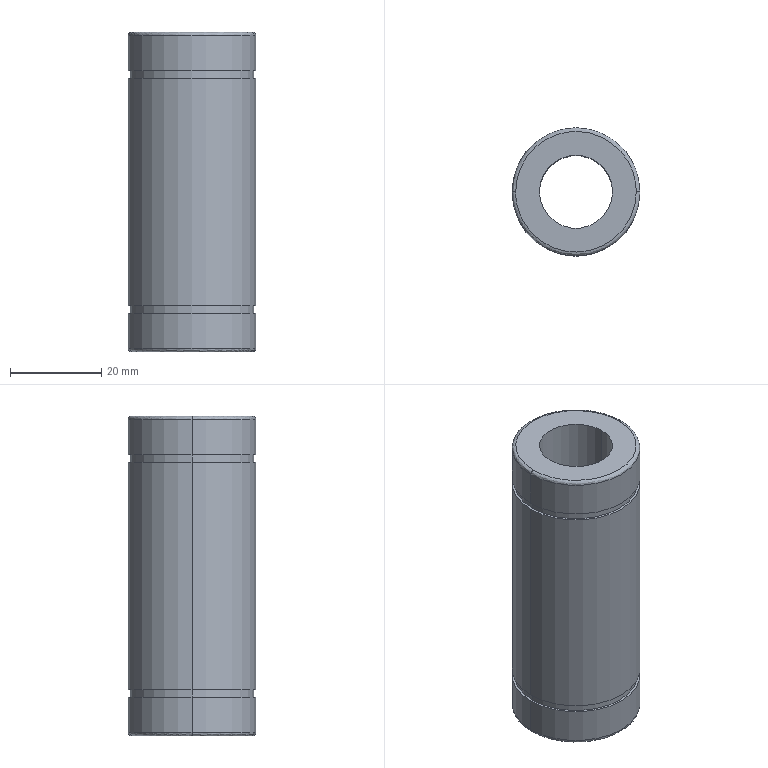Component | SolidWorks | 16mmLinearBearingSnapRingTypeLmuwm16_2_03-1 | 1 solid | 22 faces | box 28 x 28 x 70 mm | volume 28867 mm3 | cylinder 12 | plane 6 | spline 4 | commonest cylinder face diameters 28 x6 27 x4 16 x2
STEP:
#1=COLOUR_RGB('',0.7922,0.8196,0.9333);
#2=FILL_AREA_STYLE_COLOUR('',#1);
#3=FILL_AREA_STYLE('',(#2));
#4=SURFACE_STYLE_FILL_AREA(#3);
#5=SURFACE_SIDE_STYLE('',(#4));
#6=SURFACE_STYLE_USAGE(.BOTH.,#5);
#7=PRESENTATION_STYLE_ASSIGNMENT((#6));
#8=CARTESIAN_POINT('',(-24.544,-4.877,98.268));
#9=VERTEX_POINT('',#8);
#10=CARTESIAN_POINT('',(-25.583,-4.877,98.268));
#11=VERTEX_POINT('',#10);
#12=CARTESIAN_POINT('',(-24.544,-4.877,98.268));
#13=CARTESIAN_POINT('',(-24.544,-5.916,98.268));
#14=CARTESIAN_POINT('',(-25.583,-5.916,98.268));
#15=CARTESIAN_POINT('',(-25.583,-4.877,98.268));
#16=(BOUNDED_CURVE()B_SPLINE_CURVE(3,(#12,#13,#14,#15),.UNSPECIFIED.,.F.,.F.)B_SPLINE_CURVE_WITH_KNOTS((4,4),(0.,1.),.UNSPECIFIED.)CURVE()GEOMETRIC_REPRESENTATION_ITEM()RATIONAL_B_SPLINE_CURVE((1.,0.3333,0.3333,1.))REPRESENTATION_ITEM(''));
#17=EDGE_CURVE('',#9,#11,#16,.T.);
#18=ORIENTED_EDGE('',*,*,#17,.T.);
#19=CARTESIAN_POINT('',(-25.615,-4.877,98.236));
#20=VERTEX_POINT('',#19);
#21=CARTESIAN_POINT('',(-25.583,-4.877,98.236));
#22=DIRECTION('',(-0.,-1.,0.));
#23=DIRECTION('',(-1.,0.,0.));
#24=AXIS2_PLACEMENT_3D('',#21,#22,#23);
#25=CIRCLE('',#24,0.0315);
#26=EDGE_CURVE('',#11,#20,#25,.T.);
#27=ORIENTED_EDGE('',*,*,#26,.T.);
#28=CARTESIAN_POINT('',(-24.512,-4.877,98.236));
#29=VERTEX_POINT('',#28);
#30=CARTESIAN_POINT('',(-25.063,-4.877,98.236));
#31=DIRECTION('',(0.,0.,-1.));
#32=DIRECTION('',(-1.,0.,0.));
#33=AXIS2_PLACEMENT_3D('',#30,#31,#32);
#34=CIRCLE('',#33,0.5512);
#35=EDGE_CURVE('',#29,#20,#34,.T.);
#36=ORIENTED_EDGE('',*,*,#35,.F.);
#37=CARTESIAN_POINT('',(-24.544,-4.877,98.236));
#38=DIRECTION('',(0.,1.,0.));
#39=DIRECTION('',(1.,0.,0.));
#40=AXIS2_PLACEMENT_3D('',#37,#38,#39);
#41=CIRCLE('',#40,0.0315);
#42=EDGE_CURVE('',#9,#29,#41,.T.);
#43=ORIENTED_EDGE('',*,*,#42,.F.);
#44=EDGE_LOOP('',(#18,#27,#36,#43));
#45=FACE_OUTER_BOUND('',#44,.T.);
#46=CARTESIAN_POINT('',(-25.583,-4.877,98.268));
#47=CARTESIAN_POINT('',(-25.583,-5.916,98.268));
#48=CARTESIAN_POINT('',(-24.544,-5.916,98.268));
#49=CARTESIAN_POINT('',(-24.544,-4.877,98.268));
#50=CARTESIAN_POINT('',(-25.602,-4.877,98.268));
#51=CARTESIAN_POINT('',(-25.602,-5.953,98.268));
#52=CARTESIAN_POINT('',(-24.525,-5.953,98.268));
#53=CARTESIAN_POINT('',(-24.525,-4.877,98.268));
#54=CARTESIAN_POINT('',(-25.615,-4.877,98.255));
#55=CARTESIAN_POINT('',(-25.615,-5.979,98.255));
#56=CARTESIAN_POINT('',(-24.512,-5.979,98.255));
#57=CARTESIAN_POINT('',(-24.512,-4.877,98.255));
#58=CARTESIAN_POINT('',(-25.615,-4.877,98.236));
#59=CARTESIAN_POINT('',(-25.615,-5.979,98.236));
#60=CARTESIAN_POINT('',(-24.512,-5.979,98.236));
#61=CARTESIAN_POINT('',(-24.512,-4.877,98.236));
#62=(BOUNDED_SURFACE()B_SPLINE_SURFACE(3,3,((#46,#47,#48,#49),(#50,#51,#52,#53),(#54,#55,#56,#57),(#58,#59,#60,#61)),.UNSPECIFIED.,.F.,.F.,.T.)B_SPLINE_SURFACE_WITH_KNOTS((4,4),(4,4),(0.,1.),(0.,1.),.UNSPECIFIED.)GEOMETRIC_REPRESENTATION_ITEM()RATIONAL_B_SPLINE_SURFACE(((1.,0.3333,0.3333,1.),(0.8047,0.2682,0.2682,0.8047),(0.8047,0.2682,0.2682,0.8047),(1.,0.3333,0.3333,1.)))REPRESENTATION_ITEM('')SURFACE());
#63=ADVANCED_FACE('',(#45),#62,.T.);
#64=CARTESIAN_POINT('',(-25.615,-4.877,95.543));
#65=VERTEX_POINT('',#64);
#66=CARTESIAN_POINT('',(-24.512,-4.877,95.543));
#67=VERTEX_POINT('',#66);
#68=CARTESIAN_POINT('',(-25.063,-4.877,95.543));
#69=DIRECTION('',(0.,0.,1.));
#70=DIRECTION('',(-1.,0.,0.));
#71=AXIS2_PLACEMENT_3D('',#68,#69,#70);
#72=CIRCLE('',#71,0.5512);
#73=EDGE_CURVE('',#65,#67,#72,.T.);
#74=ORIENTED_EDGE('',*,*,#73,.F.);
#75=CARTESIAN_POINT('',(-25.583,-4.877,95.512));
#76=VERTEX_POINT('',#75);
#77=CARTESIAN_POINT('',(-25.583,-4.877,95.543));
#78=DIRECTION('',(-0.,-1.,0.));
#79=DIRECTION('',(-1.,0.,0.));
#80=AXIS2_PLACEMENT_3D('',#77,#78,#79);
#81=CIRCLE('',#80,0.0315);
#82=EDGE_CURVE('',#65,#76,#81,.T.);
#83=ORIENTED_EDGE('',*,*,#82,.T.);
#84=CARTESIAN_POINT('',(-24.544,-4.877,95.512));
#85=VERTEX_POINT('',#84);
#86=CARTESIAN_POINT('',(-25.583,-4.877,95.512));
#87=CARTESIAN_POINT('',(-25.583,-5.916,95.512));
#88=CARTESIAN_POINT('',(-24.544,-5.916,95.512));
#89=CARTESIAN_POINT('',(-24.544,-4.877,95.512));
#90=(BOUNDED_CURVE()B_SPLINE_CURVE(3,(#86,#87,#88,#89),.UNSPECIFIED.,.F.,.F.)B_SPLINE_CURVE_WITH_KNOTS((4,4),(0.,1.),.UNSPECIFIED.)CURVE()GEOMETRIC_REPRESENTATION_ITEM()RATIONAL_B_SPLINE_CURVE((1.,0.3333,0.3333,1.))REPRESENTATION_ITEM(''));
#91=EDGE_CURVE('',#76,#85,#90,.T.);
#92=ORIENTED_EDGE('',*,*,#91,.T.);
#93=CARTESIAN_POINT('',(-24.544,-4.877,95.543));
#94=DIRECTION('',(0.,1.,0.));
#95=DIRECTION('',(1.,0.,0.));
#96=AXIS2_PLACEMENT_3D('',#93,#94,#95);
#97=CIRCLE('',#96,0.0315);
#98=EDGE_CURVE('',#67,#85,#97,.T.);
#99=ORIENTED_EDGE('',*,*,#98,.F.);
#100=EDGE_LOOP('',(#74,#83,#92,#99));
#101=FACE_OUTER_BOUND('',#100,.T.);
#102=CARTESIAN_POINT('',(-25.615,-4.877,95.543));
#103=CARTESIAN_POINT('',(-25.615,-5.979,95.543));
#104=CARTESIAN_POINT('',(-24.512,-5.979,95.543));
#105=CARTESIAN_POINT('',(-24.512,-4.877,95.543));
#106=CARTESIAN_POINT('',(-25.615,-4.877,95.525));
#107=CARTESIAN_POINT('',(-25.615,-5.979,95.525));
#108=CARTESIAN_POINT('',(-24.512,-5.979,95.525));
#109=CARTESIAN_POINT('',(-24.512,-4.877,95.525));
#110=CARTESIAN_POINT('',(-25.602,-4.877,95.512));
#111=CARTESIAN_POINT('',(-25.602,-5.953,95.512));
#112=CARTESIAN_POINT('',(-24.525,-5.953,95.512));
#113=CARTESIAN_POINT('',(-24.525,-4.877,95.512));
#114=CARTESIAN_POINT('',(-25.583,-4.877,95.512));
#115=CARTESIAN_POINT('',(-25.583,-5.916,95.512));
#116=CARTESIAN_POINT('',(-24.544,-5.916,95.512));
#117=CARTESIAN_POINT('',(-24.544,-4.877,95.512));
#118=(BOUNDED_SURFACE()B_SPLINE_SURFACE(3,3,((#102,#103,#104,#105),(#106,#107,#108,#109),(#110,#111,#112,#113),(#114,#115,#116,#117)),.UNSPECIFIED.,.F.,.F.,.T.)B_SPLINE_SURFACE_WITH_KNOTS((4,4),(4,4),(0.,1.),(0.,1.),.UNSPECIFIED.)GEOMETRIC_REPRESENTATION_ITEM()RATIONAL_B_SPLINE_SURFACE(((1.,0.3333,0.3333,1.),(0.8047,0.2682,0.2682,0.8047),(0.8047,0.2682,0.2682,0.8047),(1.,0.3333,0.3333,1.)))REPRESENTATION_ITEM('')SURFACE());
#119=ADVANCED_FACE('',(#101),#118,.T.);
#120=CARTESIAN_POINT('',(-25.615,-4.877,97.87));
#121=VERTEX_POINT('',#120);
#122=CARTESIAN_POINT('',(-24.512,-4.877,97.87));
#123=VERTEX_POINT('',#122);
#124=CARTESIAN_POINT('',(-25.063,-4.877,97.87));
#125=DIRECTION('',(0.,0.,-1.));
#126=DIRECTION('',(-1.,0.,0.));
#127=AXIS2_PLACEMENT_3D('',#124,#125,#126);
#128=CIRCLE('',#127,0.5512);
#129=EDGE_CURVE('',#121,#123,#128,.T.);
#130=ORIENTED_EDGE('',*,*,#129,.T.);
#131=CARTESIAN_POINT('',(-24.512,-4.877,95.909));
#132=VERTEX_POINT('',#131);
#133=CARTESIAN_POINT('',(-24.512,-4.877,96.89));
#134=DIRECTION('',(0.,0.,-1.));
#135=VECTOR('',#134,39.37);
#136=LINE('',#133,#135);
#137=EDGE_CURVE('',#123,#132,#136,.T.);
#138=ORIENTED_EDGE('',*,*,#137,.T.);
#139=CARTESIAN_POINT('',(-25.615,-4.877,95.909));
#140=VERTEX_POINT('',#139);
#141=CARTESIAN_POINT('',(-25.063,-4.877,95.909));
#142=DIRECTION('',(0.,0.,1.));
#143=DIRECTION('',(-1.,0.,0.));
#144=AXIS2_PLACEMENT_3D('',#141,#142,#143);
#145=CIRCLE('',#144,0.5512);
#146=EDGE_CURVE('',#132,#140,#145,.T.);
#147=ORIENTED_EDGE('',*,*,#146,.T.);
#148=CARTESIAN_POINT('',(-25.615,-4.877,96.89));
#149=DIRECTION('',(0.,0.,-1.));
#150=VECTOR('',#149,39.37);
#151=LINE('',#148,#150);
#152=EDGE_CURVE('',#121,#140,#151,.T.);
#153=ORIENTED_EDGE('',*,*,#152,.F.);
#154=EDGE_LOOP('',(#130,#138,#147,#153));
#155=FACE_OUTER_BOUND('',#154,.T.);
#156=CARTESIAN_POINT('',(-25.063,-4.877,96.89));
#157=DIRECTION('',(0.,0.,-1.));
#158=DIRECTION('',(-1.,0.,0.));
#159=AXIS2_PLACEMENT_3D('',#156,#157,#158);
#160=CYLINDRICAL_SURFACE('',#159,0.5512);
#161=ADVANCED_FACE('',(#155),#160,.T.);
#162=CARTESIAN_POINT('',(-25.595,-4.877,97.933));
#163=VERTEX_POINT('',#162);
#164=CARTESIAN_POINT('',(-24.532,-4.877,97.933));
#165=VERTEX_POINT('',#164);
#166=CARTESIAN_POINT('',(-25.063,-4.877,97.933));
#167=DIRECTION('',(0.,0.,-1.));
#168=DIRECTION('',(-1.,0.,0.));
#169=AXIS2_PLACEMENT_3D('',#166,#167,#168);
#170=CIRCLE('',#169,0.5315);
#171=EDGE_CURVE('',#163,#165,#170,.T.);
#172=ORIENTED_EDGE('',*,*,#171,.T.);
#173=CARTESIAN_POINT('',(-24.532,-4.877,97.87));
#174=VERTEX_POINT('',#173);
#175=CARTESIAN_POINT('',(-24.532,-4.877,97.902));
#176=DIRECTION('',(0.,0.,-1.));
#177=VECTOR('',#176,39.37);
#178=LINE('',#175,#177);
#179=EDGE_CURVE('',#165,#174,#178,.T.);
#180=ORIENTED_EDGE('',*,*,#179,.T.);
#181=CARTESIAN_POINT('',(-25.595,-4.877,97.87));
#182=VERTEX_POINT('',#181);
#183=CARTESIAN_POINT('',(-25.063,-4.877,97.87));
#184=DIRECTION('',(0.,0.,-1.));
#185=DIRECTION('',(-1.,0.,0.));
#186=AXIS2_PLACEMENT_3D('',#183,#184,#185);
#187=CIRCLE('',#186,0.5315);
#188=EDGE_CURVE('',#182,#174,#187,.T.);
#189=ORIENTED_EDGE('',*,*,#188,.F.);
#190=CARTESIAN_POINT('',(-25.595,-4.877,97.902));
#191=DIRECTION('',(0.,0.,-1.));
#192=VECTOR('',#191,39.37);
#193=LINE('',#190,#192);
#194=EDGE_CURVE('',#163,#182,#193,.T.);
#195=ORIENTED_EDGE('',*,*,#194,.F.);
#196=EDGE_LOOP('',(#172,#180,#189,#195));
#197=FACE_OUTER_BOUND('',#196,.T.);
#198=CARTESIAN_POINT('',(-25.063,-4.877,97.902));
#199=DIRECTION('',(0.,0.,-1.));
#200=DIRECTION('',(-1.,0.,0.));
#201=AXIS2_PLACEMENT_3D('',#198,#199,#200);
#202=CYLINDRICAL_SURFACE('',#201,0.5315);
#203=ADVANCED_FACE('',(#197),#202,.T.);
#204=CARTESIAN_POINT('',(-24.532,-4.877,95.909));
#205=VERTEX_POINT('',#204);
#206=CARTESIAN_POINT('',(-25.595,-4.877,95.909));
#207=VERTEX_POINT('',#206);
#208=CARTESIAN_POINT('',(-25.063,-4.877,95.909));
#209=DIRECTION('',(0.,0.,1.));
#210=DIRECTION('',(-1.,0.,0.));
#211=AXIS2_PLACEMENT_3D('',#208,#209,#210);
#212=CIRCLE('',#211,0.5315);
#213=EDGE_CURVE('',#205,#207,#212,.T.);
#214=ORIENTED_EDGE('',*,*,#213,.F.);
#215=CARTESIAN_POINT('',(-24.532,-4.877,95.846));
#216=VERTEX_POINT('',#215);
#217=CARTESIAN_POINT('',(-24.532,-4.877,95.878));
#218=DIRECTION('',(0.,0.,-1.));
#219=VECTOR('',#218,39.37);
#220=LINE('',#217,#219);
#221=EDGE_CURVE('',#205,#216,#220,.T.);
#222=ORIENTED_EDGE('',*,*,#221,.T.);
#223=CARTESIAN_POINT('',(-25.595,-4.877,95.846));
#224=VERTEX_POINT('',#223);
#225=CARTESIAN_POINT('',(-25.063,-4.877,95.846));
#226=DIRECTION('',(0.,0.,1.));
#227=DIRECTION('',(-1.,0.,0.));
#228=AXIS2_PLACEMENT_3D('',#225,#226,#227);
#229=CIRCLE('',#228,0.5315);
#230=EDGE_CURVE('',#216,#224,#229,.T.);
#231=ORIENTED_EDGE('',*,*,#230,.T.);
#232=CARTESIAN_POINT('',(-25.595,-4.877,95.878));
#233=DIRECTION('',(0.,0.,-1.));
#234=VECTOR('',#233,39.37);
#235=LINE('',#232,#234);
#236=EDGE_CURVE('',#207,#224,#235,.T.);
#237=ORIENTED_EDGE('',*,*,#236,.F.);
#238=EDGE_LOOP('',(#214,#222,#231,#237));
#239=FACE_OUTER_BOUND('',#238,.T.);
#240=CARTESIAN_POINT('',(-25.063,-4.877,95.878));
#241=DIRECTION('',(0.,0.,-1.));
#242=DIRECTION('',(-1.,0.,0.));
#243=AXIS2_PLACEMENT_3D('',#240,#241,#242);
#244=CYLINDRICAL_SURFACE('',#243,0.5315);
#245=ADVANCED_FACE('',(#239),#244,.T.);
#246=CARTESIAN_POINT('',(-25.063,-4.877,98.236));
#247=DIRECTION('',(0.,0.,-1.));
#248=DIRECTION('',(-1.,0.,0.));
#249=AXIS2_PLACEMENT_3D('',#246,#247,#248);
#250=CIRCLE('',#249,0.5512);
#251=EDGE_CURVE('',#20,#29,#250,.T.);
#252=ORIENTED_EDGE('',*,*,#251,.T.);
#253=CARTESIAN_POINT('',(-24.512,-4.877,97.933));
#254=VERTEX_POINT('',#253);
#255=CARTESIAN_POINT('',(-24.512,-4.877,98.085));
#256=DIRECTION('',(0.,0.,-1.));
#257=VECTOR('',#256,39.37);
#258=LINE('',#255,#257);
#259=EDGE_CURVE('',#29,#254,#258,.T.);
#260=ORIENTED_EDGE('',*,*,#259,.T.);
#261=CARTESIAN_POINT('',(-25.615,-4.877,97.933));
#262=VERTEX_POINT('',#261);
#263=CARTESIAN_POINT('',(-25.063,-4.877,97.933));
#264=DIRECTION('',(0.,0.,-1.));
#265=DIRECTION('',(-1.,0.,0.));
#266=AXIS2_PLACEMENT_3D('',#263,#264,#265);
#267=CIRCLE('',#266,0.5512);
#268=EDGE_CURVE('',#262,#254,#267,.T.);
#269=ORIENTED_EDGE('',*,*,#268,.F.);
#270=CARTESIAN_POINT('',(-25.615,-4.877,98.085));
#271=DIRECTION('',(0.,0.,-1.));
#272=VECTOR('',#271,39.37);
#273=LINE('',#270,#272);
#274=EDGE_CURVE('',#20,#262,#273,.T.);
#275=ORIENTED_EDGE('',*,*,#274,.F.);
#276=EDGE_LOOP('',(#252,#260,#269,#275));
#277=FACE_OUTER_BOUND('',#276,.T.);
#278=CARTESIAN_POINT('',(-25.063,-4.877,98.085));
#279=DIRECTION('',(0.,0.,-1.));
#280=DIRECTION('',(-1.,0.,0.));
#281=AXIS2_PLACEMENT_3D('',#278,#279,#280);
#282=CYLINDRICAL_SURFACE('',#281,0.5512);
#283=ADVANCED_FACE('',(#277),#282,.T.);
#284=CARTESIAN_POINT('',(-24.512,-4.877,95.846));
#285=VERTEX_POINT('',#284);
#286=CARTESIAN_POINT('',(-25.615,-4.877,95.846));
#287=VERTEX_POINT('',#286);
#288=CARTESIAN_POINT('',(-25.063,-4.877,95.846));
#289=DIRECTION('',(0.,0.,1.));
#290=DIRECTION('',(-1.,0.,0.));
#291=AXIS2_PLACEMENT_3D('',#288,#289,#290);
#292=CIRCLE('',#291,0.5512);
#293=EDGE_CURVE('',#285,#287,#292,.T.);
#294=ORIENTED_EDGE('',*,*,#293,.F.);
#295=CARTESIAN_POINT('',(-24.512,-4.877,95.695));
#296=DIRECTION('',(0.,0.,-1.));
#297=VECTOR('',#296,39.37);
#298=LINE('',#295,#297);
#299=EDGE_CURVE('',#285,#67,#298,.T.);
#300=ORIENTED_EDGE('',*,*,#299,.T.);
#301=CARTESIAN_POINT('',(-25.063,-4.877,95.543));
#302=DIRECTION('',(0.,0.,1.));
#303=DIRECTION('',(-1.,0.,0.));
#304=AXIS2_PLACEMENT_3D('',#301,#302,#303);
#305=CIRCLE('',#304,0.5512);
#306=EDGE_CURVE('',#67,#65,#305,.T.);
#307=ORIENTED_EDGE('',*,*,#306,.T.);
#308=CARTESIAN_POINT('',(-25.615,-4.877,95.695));
#309=DIRECTION('',(0.,0.,-1.));
#310=VECTOR('',#309,39.37);
#311=LINE('',#308,#310);
#312=EDGE_CURVE('',#287,#65,#311,.T.);
#313=ORIENTED_EDGE('',*,*,#312,.F.);
#314=EDGE_LOOP('',(#294,#300,#307,#313));
#315=FACE_OUTER_BOUND('',#314,.T.);
#316=CARTESIAN_POINT('',(-25.063,-4.877,95.695));
#317=DIRECTION('',(0.,0.,-1.));
#318=DIRECTION('',(-1.,0.,0.));
#319=AXIS2_PLACEMENT_3D('',#316,#317,#318);
#320=CYLINDRICAL_SURFACE('',#319,0.5512);
#321=ADVANCED_FACE('',(#315),#320,.T.);
#322=CARTESIAN_POINT('',(-24.749,-4.877,98.268));
#323=VERTEX_POINT('',#322);
#324=CARTESIAN_POINT('',(-25.378,-4.877,98.268));
#325=VERTEX_POINT('',#324);
#326=CARTESIAN_POINT('',(-25.063,-4.877,98.268));
#327=DIRECTION('',(0.,0.,-1.));
#328=DIRECTION('',(-1.,0.,0.));
#329=AXIS2_PLACEMENT_3D('',#326,#327,#328);
#330=CIRCLE('',#329,0.315);
#331=EDGE_CURVE('',#323,#325,#330,.T.);
#332=ORIENTED_EDGE('',*,*,#331,.F.);
#333=CARTESIAN_POINT('',(-24.749,-4.877,95.512));
#334=VERTEX_POINT('',#333);
#335=CARTESIAN_POINT('',(-24.749,-4.877,96.89));
#336=DIRECTION('',(0.,0.,-1.));
#337=VECTOR('',#336,39.37);
#338=LINE('',#335,#337);
#339=EDGE_CURVE('',#323,#334,#338,.T.);
#340=ORIENTED_EDGE('',*,*,#339,.T.);
#341=CARTESIAN_POINT('',(-25.378,-4.877,95.512));
#342=VERTEX_POINT('',#341);
#343=CARTESIAN_POINT('',(-25.063,-4.877,95.512));
#344=DIRECTION('',(0.,0.,1.));
#345=DIRECTION('',(-1.,0.,0.));
#346=AXIS2_PLACEMENT_3D('',#343,#344,#345);
#347=CIRCLE('',#346,0.315);
#348=EDGE_CURVE('',#342,#334,#347,.T.);
#349=ORIENTED_EDGE('',*,*,#348,.F.);
#350=CARTESIAN_POINT('',(-25.378,-4.877,96.89));
#351=DIRECTION('',(0.,0.,-1.));
#352=VECTOR('',#351,39.37);
#353=LINE('',#350,#352);
#354=EDGE_CURVE('',#325,#342,#353,.T.);
#355=ORIENTED_EDGE('',*,*,#354,.F.);
#356=EDGE_LOOP('',(#332,#340,#349,#355));
#357=FACE_OUTER_BOUND('',#356,.T.);
#358=CARTESIAN_POINT('',(-25.063,-4.877,96.89));
#359=DIRECTION('',(0.,0.,-1.));
#360=DIRECTION('',(-1.,0.,0.));
#361=AXIS2_PLACEMENT_3D('',#358,#359,#360);
#362=CYLINDRICAL_SURFACE('',#361,0.315);
#363=ADVANCED_FACE('',(#357),#362,.F.);
#364=ORIENTED_EDGE('',*,*,#137,.F.);
#365=CARTESIAN_POINT('',(-25.063,-4.877,97.87));
#366=DIRECTION('',(0.,0.,-1.));
#367=DIRECTION('',(-1.,0.,0.));
#368=AXIS2_PLACEMENT_3D('',#365,#366,#367);
#369=CIRCLE('',#368,0.5512);
#370=EDGE_CURVE('',#123,#121,#369,.T.);
#371=ORIENTED_EDGE('',*,*,#370,.T.);
#372=ORIENTED_EDGE('',*,*,#152,.T.);
#373=CARTESIAN_POINT('',(-25.063,-4.877,95.909));
#374=DIRECTION('',(0.,0.,1.));
#375=DIRECTION('',(-1.,0.,0.));
#376=AXIS2_PLACEMENT_3D('',#373,#374,#375);
#377=CIRCLE('',#376,0.5512);
#378=EDGE_CURVE('',#140,#132,#377,.T.);
#379=ORIENTED_EDGE('',*,*,#378,.T.);
#380=EDGE_LOOP('',(#364,#371,#372,#379));
#381=FACE_OUTER_BOUND('',#380,.T.);
#382=CARTESIAN_POINT('',(-25.063,-4.877,96.89));
#383=DIRECTION('',(0.,0.,-1.));
#384=DIRECTION('',(-1.,0.,0.));
#385=AXIS2_PLACEMENT_3D('',#382,#383,#384);
#386=CYLINDRICAL_SURFACE('',#385,0.5512);
#387=ADVANCED_FACE('',(#381),#386,.T.);
#388=ORIENTED_EDGE('',*,*,#129,.F.);
#389=ORIENTED_EDGE('',*,*,#370,.F.);
#390=EDGE_LOOP('',(#388,#389));
#391=FACE_OUTER_BOUND('',#390,.T.);
#392=ORIENTED_EDGE('',*,*,#188,.T.);
#393=CARTESIAN_POINT('',(-25.063,-4.877,97.87));
#394=DIRECTION('',(0.,0.,-1.));
#395=DIRECTION('',(-1.,0.,0.));
#396=AXIS2_PLACEMENT_3D('',#393,#394,#395);
#397=CIRCLE('',#396,0.5315);
#398=EDGE_CURVE('',#174,#182,#397,.T.);
#399=ORIENTED_EDGE('',*,*,#398,.T.);
#400=EDGE_LOOP('',(#392,#399));
#401=FACE_BOUND('',#400,.T.);
#402=CARTESIAN_POINT('',(-25.063,-4.336,97.87));
#403=DIRECTION('',(0.,0.,1.));
#404=DIRECTION('',(1.,0.,0.));
#405=AXIS2_PLACEMENT_3D('',#402,#403,#404);
#406=PLANE('',#405);
#407=ADVANCED_FACE('',(#391,#401),#406,.T.);
#408=CARTESIAN_POINT('',(-25.063,-4.877,95.909));
#409=DIRECTION('',(0.,0.,1.));
#410=DIRECTION('',(-1.,0.,0.));
#411=AXIS2_PLACEMENT_3D('',#408,#409,#410);
#412=CIRCLE('',#411,0.5315);
#413=EDGE_CURVE('',#207,#205,#412,.T.);
#414=ORIENTED_EDGE('',*,*,#413,.T.);
#415=ORIENTED_EDGE('',*,*,#213,.T.);
#416=EDGE_LOOP('',(#414,#415));
#417=FACE_BOUND('',#416,.T.);
#418=ORIENTED_EDGE('',*,*,#378,.F.);
#419=ORIENTED_EDGE('',*,*,#146,.F.);
#420=EDGE_LOOP('',(#418,#419));
#421=FACE_OUTER_BOUND('',#420,.T.);
#422=CARTESIAN_POINT('',(-25.063,-4.336,95.909));
#423=DIRECTION('',(0.,0.,-1.));
#424=DIRECTION('',(-1.,0.,0.));
#425=AXIS2_PLACEMENT_3D('',#422,#423,#424);
#426=PLANE('',#425);
#427=ADVANCED_FACE('',(#417,#421),#426,.T.);
#428=ORIENTED_EDGE('',*,*,#179,.F.);
#429=CARTESIAN_POINT('',(-25.063,-4.877,97.933));
#430=DIRECTION('',(0.,0.,-1.));
#431=DIRECTION('',(-1.,0.,0.));
#432=AXIS2_PLACEMENT_3D('',#429,#430,#431);
#433=CIRCLE('',#432,0.5315);
#434=EDGE_CURVE('',#165,#163,#433,.T.);
#435=ORIENTED_EDGE('',*,*,#434,.T.);
#436=ORIENTED_EDGE('',*,*,#194,.T.);
#437=ORIENTED_EDGE('',*,*,#398,.F.);
#438=EDGE_LOOP('',(#428,#435,#436,#437));
#439=FACE_OUTER_BOUND('',#438,.T.);
#440=CARTESIAN_POINT('',(-25.063,-4.877,97.902));
#441=DIRECTION('',(0.,0.,-1.));
#442=DIRECTION('',(-1.,0.,0.));
#443=AXIS2_PLACEMENT_3D('',#440,#441,#442);
#444=CYLINDRICAL_SURFACE('',#443,0.5315);
#445=ADVANCED_FACE('',(#439),#444,.T.);
#446=ORIENTED_EDGE('',*,*,#221,.F.);
#447=ORIENTED_EDGE('',*,*,#413,.F.);
#448=ORIENTED_EDGE('',*,*,#236,.T.);
#449=CARTESIAN_POINT('',(-25.063,-4.877,95.846));
#450=DIRECTION('',(0.,0.,1.));
#451=DIRECTION('',(-1.,0.,0.));
#452=AXIS2_PLACEMENT_3D('',#449,#450,#451);
#453=CIRCLE('',#452,0.5315);
#454=EDGE_CURVE('',#224,#216,#453,.T.);
#455=ORIENTED_EDGE('',*,*,#454,.T.);
#456=EDGE_LOOP('',(#446,#447,#448,#455));
#457=FACE_OUTER_BOUND('',#456,.T.);
#458=CARTESIAN_POINT('',(-25.063,-4.877,95.878));
#459=DIRECTION('',(0.,0.,-1.));
#460=DIRECTION('',(-1.,0.,0.));
#461=AXIS2_PLACEMENT_3D('',#458,#459,#460);
#462=CYLINDRICAL_SURFACE('',#461,0.5315);
#463=ADVANCED_FACE('',(#457),#462,.T.);
#464=ORIENTED_EDGE('',*,*,#171,.F.);
#465=ORIENTED_EDGE('',*,*,#434,.F.);
#466=EDGE_LOOP('',(#464,#465));
#467=FACE_BOUND('',#466,.T.);
#468=ORIENTED_EDGE('',*,*,#268,.T.);
#469=CARTESIAN_POINT('',(-25.063,-4.877,97.933));
#470=DIRECTION('',(0.,0.,-1.));
#471=DIRECTION('',(-1.,0.,0.));
#472=AXIS2_PLACEMENT_3D('',#469,#470,#471);
#473=CIRCLE('',#472,0.5512);
#474=EDGE_CURVE('',#254,#262,#473,.T.);
#475=ORIENTED_EDGE('',*,*,#474,.T.);
#476=EDGE_LOOP('',(#468,#475));
#477=FACE_OUTER_BOUND('',#476,.T.);
#478=CARTESIAN_POINT('',(-25.063,-4.336,97.933));
#479=DIRECTION('',(0.,0.,-1.));
#480=DIRECTION('',(-1.,0.,0.));
#481=AXIS2_PLACEMENT_3D('',#478,#479,#480);
#482=PLANE('',#481);
#483=ADVANCED_FACE('',(#467,#477),#482,.T.);
#484=CARTESIAN_POINT('',(-25.063,-4.877,95.846));
#485=DIRECTION('',(0.,0.,1.));
#486=DIRECTION('',(-1.,0.,0.));
#487=AXIS2_PLACEMENT_3D('',#484,#485,#486);
#488=CIRCLE('',#487,0.5512);
#489=EDGE_CURVE('',#287,#285,#488,.T.);
#490=ORIENTED_EDGE('',*,*,#489,.T.);
#491=ORIENTED_EDGE('',*,*,#293,.T.);
#492=EDGE_LOOP('',(#490,#491));
#493=FACE_OUTER_BOUND('',#492,.T.);
#494=ORIENTED_EDGE('',*,*,#454,.F.);
#495=ORIENTED_EDGE('',*,*,#230,.F.);
#496=EDGE_LOOP('',(#494,#495));
#497=FACE_BOUND('',#496,.T.);
#498=CARTESIAN_POINT('',(-25.063,-4.336,95.846));
#499=DIRECTION('',(0.,0.,1.));
#500=DIRECTION('',(1.,0.,0.));
#501=AXIS2_PLACEMENT_3D('',#498,#499,#500);
#502=PLANE('',#501);
#503=ADVANCED_FACE('',(#493,#497),#502,.T.);
#504=ORIENTED_EDGE('',*,*,#259,.F.);
#505=ORIENTED_EDGE('',*,*,#35,.T.);
#506=ORIENTED_EDGE('',*,*,#274,.T.);
#507=ORIENTED_EDGE('',*,*,#474,.F.);
#508=EDGE_LOOP('',(#504,#505,#506,#507));
#509=FACE_OUTER_BOUND('',#508,.T.);
#510=CARTESIAN_POINT('',(-25.063,-4.877,98.085));
#511=DIRECTION('',(0.,0.,-1.));
#512=DIRECTION('',(-1.,0.,0.));
#513=AXIS2_PLACEMENT_3D('',#510,#511,#512);
#514=CYLINDRICAL_SURFACE('',#513,0.5512);
#515=ADVANCED_FACE('',(#509),#514,.T.);
#516=ORIENTED_EDGE('',*,*,#299,.F.);
#517=ORIENTED_EDGE('',*,*,#489,.F.);
#518=ORIENTED_EDGE('',*,*,#312,.T.);
#519=ORIENTED_EDGE('',*,*,#73,.T.);
#520=EDGE_LOOP('',(#516,#517,#518,#519));
#521=FACE_OUTER_BOUND('',#520,.T.);
#522=CARTESIAN_POINT('',(-25.063,-4.877,95.695));
#523=DIRECTION('',(0.,0.,-1.));
#524=DIRECTION('',(-1.,0.,0.));
#525=AXIS2_PLACEMENT_3D('',#522,#523,#524);
#526=CYLINDRICAL_SURFACE('',#525,0.5512);
#527=ADVANCED_FACE('',(#521),#526,.T.);
#528=ORIENTED_EDGE('',*,*,#26,.F.);
#529=CARTESIAN_POINT('',(-25.063,-4.357,98.268));
#530=VERTEX_POINT('',#529);
#531=CARTESIAN_POINT('',(-25.583,-4.877,98.268));
#532=CARTESIAN_POINT('',(-25.583,-4.572,98.268));
#533=CARTESIAN_POINT('',(-25.368,-4.357,98.268));
#534=CARTESIAN_POINT('',(-25.063,-4.357,98.268));
#535=(BOUNDED_CURVE()B_SPLINE_CURVE(3,(#531,#532,#533,#534),.UNSPECIFIED.,.F.,.T.)B_SPLINE_CURVE_WITH_KNOTS((4,4),(0.,1.),.UNSPECIFIED.)CURVE()GEOMETRIC_REPRESENTATION_ITEM()RATIONAL_B_SPLINE_CURVE((1.,0.8047,0.8047,1.))REPRESENTATION_ITEM(''));
#536=EDGE_CURVE('',#11,#530,#535,.T.);
#537=ORIENTED_EDGE('',*,*,#536,.T.);
#538=CARTESIAN_POINT('',(-25.063,-4.357,98.268));
#539=CARTESIAN_POINT('',(-24.759,-4.357,98.268));
#540=CARTESIAN_POINT('',(-24.544,-4.572,98.268));
#541=CARTESIAN_POINT('',(-24.544,-4.877,98.268));
#542=(BOUNDED_CURVE()B_SPLINE_CURVE(3,(#538,#539,#540,#541),.UNSPECIFIED.,.F.,.T.)B_SPLINE_CURVE_WITH_KNOTS((4,4),(0.,1.),.UNSPECIFIED.)CURVE()GEOMETRIC_REPRESENTATION_ITEM()RATIONAL_B_SPLINE_CURVE((1.,0.8047,0.8047,1.))REPRESENTATION_ITEM(''));
#543=EDGE_CURVE('',#530,#9,#542,.T.);
#544=ORIENTED_EDGE('',*,*,#543,.T.);
#545=ORIENTED_EDGE('',*,*,#42,.T.);
#546=ORIENTED_EDGE('',*,*,#251,.F.);
#547=EDGE_LOOP('',(#528,#537,#544,#545,#546));
#548=FACE_OUTER_BOUND('',#547,.T.);
#549=CARTESIAN_POINT('',(-24.544,-4.877,98.268));
#550=CARTESIAN_POINT('',(-24.544,-3.838,98.268));
#551=CARTESIAN_POINT('',(-25.583,-3.838,98.268));
#552=CARTESIAN_POINT('',(-25.583,-4.877,98.268));
#553=CARTESIAN_POINT('',(-24.525,-4.877,98.268));
#554=CARTESIAN_POINT('',(-24.525,-3.801,98.268));
#555=CARTESIAN_POINT('',(-25.602,-3.801,98.268));
#556=CARTESIAN_POINT('',(-25.602,-4.877,98.268));
#557=CARTESIAN_POINT('',(-24.512,-4.877,98.255));
#558=CARTESIAN_POINT('',(-24.512,-3.775,98.255));
#559=CARTESIAN_POINT('',(-25.615,-3.775,98.255));
#560=CARTESIAN_POINT('',(-25.615,-4.877,98.255));
#561=CARTESIAN_POINT('',(-24.512,-4.877,98.236));
#562=CARTESIAN_POINT('',(-24.512,-3.775,98.236));
#563=CARTESIAN_POINT('',(-25.615,-3.775,98.236));
#564=CARTESIAN_POINT('',(-25.615,-4.877,98.236));
#565=(BOUNDED_SURFACE()B_SPLINE_SURFACE(3,3,((#549,#550,#551,#552),(#553,#554,#555,#556),(#557,#558,#559,#560),(#561,#562,#563,#564)),.UNSPECIFIED.,.F.,.F.,.F.)B_SPLINE_SURFACE_WITH_KNOTS((4,4),(4,4),(0.,1.),(0.,1.),.UNSPECIFIED.)GEOMETRIC_REPRESENTATION_ITEM()RATIONAL_B_SPLINE_SURFACE(((1.,0.3333,0.3333,1.),(0.8047,0.2682,0.2682,0.8047),(0.8047,0.2682,0.2682,0.8047),(1.,0.3333,0.3333,1.)))REPRESENTATION_ITEM('')SURFACE());
#566=ADVANCED_FACE('',(#548),#565,.T.);
#567=ORIENTED_EDGE('',*,*,#82,.F.);
#568=ORIENTED_EDGE('',*,*,#306,.F.);
#569=ORIENTED_EDGE('',*,*,#98,.T.);
#570=CARTESIAN_POINT('',(-25.063,-4.357,95.512));
#571=VERTEX_POINT('',#570);
#572=CARTESIAN_POINT('',(-24.544,-4.877,95.512));
#573=CARTESIAN_POINT('',(-24.544,-4.572,95.512));
#574=CARTESIAN_POINT('',(-24.759,-4.357,95.512));
#575=CARTESIAN_POINT('',(-25.063,-4.357,95.512));
#576=(BOUNDED_CURVE()B_SPLINE_CURVE(3,(#572,#573,#574,#575),.UNSPECIFIED.,.F.,.F.)B_SPLINE_CURVE_WITH_KNOTS((4,4),(0.,1.),.UNSPECIFIED.)CURVE()GEOMETRIC_REPRESENTATION_ITEM()RATIONAL_B_SPLINE_CURVE((1.,0.8047,0.8047,1.))REPRESENTATION_ITEM(''));
#577=EDGE_CURVE('',#85,#571,#576,.T.);
#578=ORIENTED_EDGE('',*,*,#577,.T.);
#579=CARTESIAN_POINT('',(-25.063,-4.357,95.512));
#580=CARTESIAN_POINT('',(-25.368,-4.357,95.512));
#581=CARTESIAN_POINT('',(-25.583,-4.572,95.512));
#582=CARTESIAN_POINT('',(-25.583,-4.877,95.512));
#583=(BOUNDED_CURVE()B_SPLINE_CURVE(3,(#579,#580,#581,#582),.UNSPECIFIED.,.F.,.F.)B_SPLINE_CURVE_WITH_KNOTS((4,4),(0.,1.),.UNSPECIFIED.)CURVE()GEOMETRIC_REPRESENTATION_ITEM()RATIONAL_B_SPLINE_CURVE((1.,0.8047,0.8047,1.))REPRESENTATION_ITEM(''));
#584=EDGE_CURVE('',#571,#76,#583,.T.);
#585=ORIENTED_EDGE('',*,*,#584,.T.);
#586=EDGE_LOOP('',(#567,#568,#569,#578,#585));
#587=FACE_OUTER_BOUND('',#586,.T.);
#588=CARTESIAN_POINT('',(-24.512,-4.877,95.543));
#589=CARTESIAN_POINT('',(-24.512,-3.775,95.543));
#590=CARTESIAN_POINT('',(-25.615,-3.775,95.543));
#591=CARTESIAN_POINT('',(-25.615,-4.877,95.543));
#592=CARTESIAN_POINT('',(-24.512,-4.877,95.525));
#593=CARTESIAN_POINT('',(-24.512,-3.775,95.525));
#594=CARTESIAN_POINT('',(-25.615,-3.775,95.525));
#595=CARTESIAN_POINT('',(-25.615,-4.877,95.525));
#596=CARTESIAN_POINT('',(-24.525,-4.877,95.512));
#597=CARTESIAN_POINT('',(-24.525,-3.801,95.512));
#598=CARTESIAN_POINT('',(-25.602,-3.801,95.512));
#599=CARTESIAN_POINT('',(-25.602,-4.877,95.512));
#600=CARTESIAN_POINT('',(-24.544,-4.877,95.512));
#601=CARTESIAN_POINT('',(-24.544,-3.838,95.512));
#602=CARTESIAN_POINT('',(-25.583,-3.838,95.512));
#603=CARTESIAN_POINT('',(-25.583,-4.877,95.512));
#604=(BOUNDED_SURFACE()B_SPLINE_SURFACE(3,3,((#588,#589,#590,#591),(#592,#593,#594,#595),(#596,#597,#598,#599),(#600,#601,#602,#603)),.UNSPECIFIED.,.F.,.F.,.T.)B_SPLINE_SURFACE_WITH_KNOTS((4,4),(4,4),(0.,1.),(0.,1.),.UNSPECIFIED.)GEOMETRIC_REPRESENTATION_ITEM()RATIONAL_B_SPLINE_SURFACE(((1.,0.3333,0.3333,1.),(0.8047,0.2682,0.2682,0.8047),(0.8047,0.2682,0.2682,0.8047),(1.,0.3333,0.3333,1.)))REPRESENTATION_ITEM('')SURFACE());
#605=ADVANCED_FACE('',(#587),#604,.T.);
#606=ORIENTED_EDGE('',*,*,#17,.F.);
#607=ORIENTED_EDGE('',*,*,#543,.F.);
#608=ORIENTED_EDGE('',*,*,#536,.F.);
#609=EDGE_LOOP('',(#606,#607,#608));
#610=FACE_OUTER_BOUND('',#609,.T.);
#611=CARTESIAN_POINT('',(-25.063,-4.877,98.268));
#612=DIRECTION('',(0.,0.,-1.));
#613=DIRECTION('',(-1.,0.,0.));
#614=AXIS2_PLACEMENT_3D('',#611,#612,#613);
#615=CIRCLE('',#614,0.315);
#616=EDGE_CURVE('',#325,#323,#615,.T.);
#617=ORIENTED_EDGE('',*,*,#616,.T.);
#618=ORIENTED_EDGE('',*,*,#331,.T.);
#619=EDGE_LOOP('',(#617,#618));
#620=FACE_BOUND('',#619,.T.);
#621=CARTESIAN_POINT('',(-25.063,-4.46,98.268));
#622=DIRECTION('',(0.,0.,1.));
#623=DIRECTION('',(1.,0.,0.));
#624=AXIS2_PLACEMENT_3D('',#621,#622,#623);
#625=PLANE('',#624);
#626=ADVANCED_FACE('',(#610,#620),#625,.T.);
#627=ORIENTED_EDGE('',*,*,#348,.T.);
#628=CARTESIAN_POINT('',(-25.063,-4.877,95.512));
#629=DIRECTION('',(0.,0.,1.));
#630=DIRECTION('',(-1.,0.,0.));
#631=AXIS2_PLACEMENT_3D('',#628,#629,#630);
#632=CIRCLE('',#631,0.315);
#633=EDGE_CURVE('',#334,#342,#632,.T.);
#634=ORIENTED_EDGE('',*,*,#633,.T.);
#635=EDGE_LOOP('',(#627,#634));
#636=FACE_BOUND('',#635,.T.);
#637=ORIENTED_EDGE('',*,*,#577,.F.);
#638=ORIENTED_EDGE('',*,*,#91,.F.);
#639=ORIENTED_EDGE('',*,*,#584,.F.);
#640=EDGE_LOOP('',(#637,#638,#639));
#641=FACE_OUTER_BOUND('',#640,.T.);
#642=CARTESIAN_POINT('',(-25.063,-4.46,95.512));
#643=DIRECTION('',(0.,0.,-1.));
#644=DIRECTION('',(-1.,0.,0.));
#645=AXIS2_PLACEMENT_3D('',#642,#643,#644);
#646=PLANE('',#645);
#647=ADVANCED_FACE('',(#636,#641),#646,.T.);
#648=ORIENTED_EDGE('',*,*,#339,.F.);
#649=ORIENTED_EDGE('',*,*,#616,.F.);
#650=ORIENTED_EDGE('',*,*,#354,.T.);
#651=ORIENTED_EDGE('',*,*,#633,.F.);
#652=EDGE_LOOP('',(#648,#649,#650,#651));
#653=FACE_OUTER_BOUND('',#652,.T.);
#654=CARTESIAN_POINT('',(-25.063,-4.877,96.89));
#655=DIRECTION('',(0.,0.,-1.));
#656=DIRECTION('',(-1.,0.,0.));
#657=AXIS2_PLACEMENT_3D('',#654,#655,#656);
#658=CYLINDRICAL_SURFACE('',#657,0.315);
#659=ADVANCED_FACE('',(#653),#658,.F.);
#660=CLOSED_SHELL('',(#63,#119,#161,#203,#245,#283,#321,#363,#387,#407,#427,#445,#463,#483,#503,#515,#527,#566,#605,#626,#647,#659));
#661=MANIFOLD_SOLID_BREP('',#660);
#662=STYLED_ITEM('',(#7),#661);
#663=(LENGTH_UNIT()NAMED_UNIT(*)SI_UNIT($,.METRE.));
#664=LENGTH_MEASURE_WITH_UNIT(LENGTH_MEASURE(0.0254),#663);
#665=DIMENSIONAL_EXPONENTS(1.,0.,0.,0.,0.,0.,0.);
#666=(CONVERSION_BASED_UNIT('',#664)LENGTH_UNIT()NAMED_UNIT(#665));
#667=UNCERTAINTY_MEASURE_WITH_UNIT(LENGTH_MEASURE(0.00001),#666,'','');
#668=(NAMED_UNIT(*)PLANE_ANGLE_UNIT()SI_UNIT($,.RADIAN.));
#669=(NAMED_UNIT(*)SI_UNIT($,.STERADIAN.)SOLID_ANGLE_UNIT());
#670=(GEOMETRIC_REPRESENTATION_CONTEXT(3)GLOBAL_UNCERTAINTY_ASSIGNED_CONTEXT((#667))GLOBAL_UNIT_ASSIGNED_CONTEXT((#666,#668,#669))REPRESENTATION_CONTEXT('',''));
#671=MECHANICAL_DESIGN_GEOMETRIC_PRESENTATION_REPRESENTATION('',(#662),#670);
#672=PRESENTATION_LAYER_ASSIGNMENT('','',(#662));
#673=CARTESIAN_POINT('',(0.,0.,0.));
#674=DIRECTION('',(0.,0.,1.));
#675=DIRECTION('',(1.,0.,0.));
#676=AXIS2_PLACEMENT_3D('',#673,#674,#675);
#677=(LENGTH_UNIT()NAMED_UNIT(*)SI_UNIT($,.METRE.));
#678=LENGTH_MEASURE_WITH_UNIT(LENGTH_MEASURE(0.0254),#677);
#679=DIMENSIONAL_EXPONENTS(1.,0.,0.,0.,0.,0.,0.);
#680=(CONVERSION_BASED_UNIT('',#678)LENGTH_UNIT()NAMED_UNIT(#679));
#681=UNCERTAINTY_MEASURE_WITH_UNIT(LENGTH_MEASURE(0.00001),#680,'','');
#682=(NAMED_UNIT(*)PLANE_ANGLE_UNIT()SI_UNIT($,.RADIAN.));
#683=(NAMED_UNIT(*)SI_UNIT($,.STERADIAN.)SOLID_ANGLE_UNIT());
#684=(GEOMETRIC_REPRESENTATION_CONTEXT(3)GLOBAL_UNCERTAINTY_ASSIGNED_CONTEXT((#681))GLOBAL_UNIT_ASSIGNED_CONTEXT((#680,#682,#683))REPRESENTATION_CONTEXT('',''));
#685=ADVANCED_BREP_SHAPE_REPRESENTATION('',(#661,#676),#684);